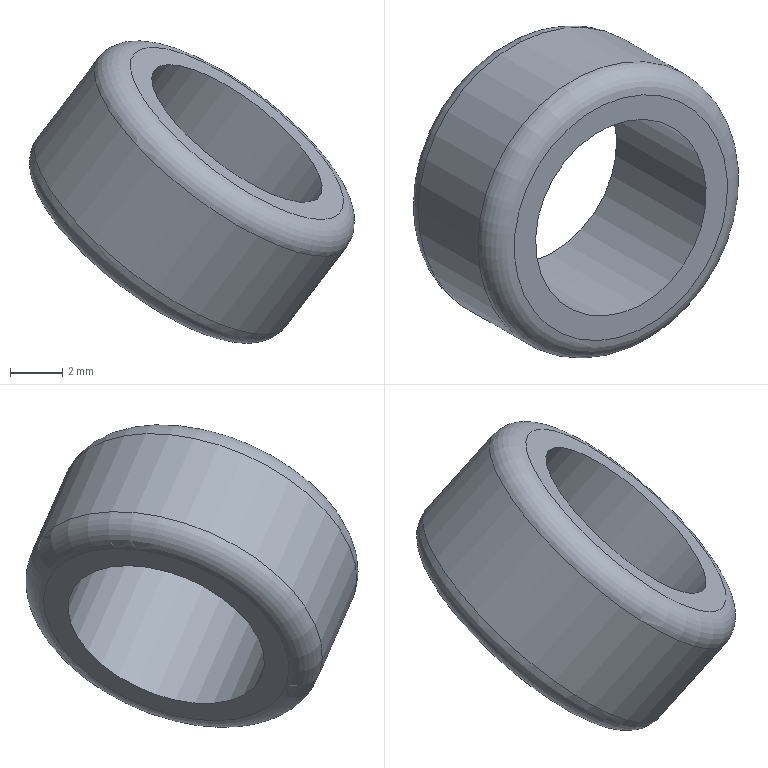Component | NX | YUAN_HUAN_KUAI | 1 solid | 6 faces | volume 361 mm3 | cylinder 2 | plane 2 | torus 2 | commonest cylinder face diameters 12 x1 8 x1
STEP:
#1=CARTESIAN_POINT('',(0.,0.,0.));
#2=DIRECTION('',(0.,0.,1.));
#3=DIRECTION('',(1.,0.,0.));
#4=AXIS2_PLACEMENT_3D('',#1,#2,#3);
#5=CARTESIAN_POINT('',(-203.835,-46.755,66.676));
#6=VERTEX_POINT('',#5);
#7=CARTESIAN_POINT('',(-201.952,-41.152,67.703));
#8=DIRECTION('',(0.5736,-0.3301,0.7497));
#9=DIRECTION('',(-0.3138,-0.9339,-0.1711));
#10=AXIS2_PLACEMENT_3D('',#7,#8,#9);
#11=CIRCLE('',#10,6.);
#12=CARTESIAN_POINT('',(-199.085,-42.802,71.452));
#13=DIRECTION('',(-0.5736,0.3301,-0.7497));
#14=DIRECTION('',(0.3138,0.9339,0.1711));
#15=AXIS2_PLACEMENT_3D('',#12,#13,#14);
#16=CYLINDRICAL_SURFACE('',#15,6.);
#17=CARTESIAN_POINT('',(9.425,5.));
#18=DIRECTION('',(-1.,0.));
#19=VECTOR('',#18,1.);
#20=LINE('',#17,#19);
#21=(GEOMETRIC_REPRESENTATION_CONTEXT(2)PARAMETRIC_REPRESENTATION_CONTEXT()REPRESENTATION_CONTEXT('',''));
#22=DEFINITIONAL_REPRESENTATION('',(#20),#21);
#23=PCURVE('',#16,#22);
#24=CARTESIAN_POINT('',(-201.952,-41.152,67.703));
#25=DIRECTION('',(0.5736,-0.3301,0.7497));
#26=DIRECTION('',(-0.3138,-0.9339,-0.1711));
#27=AXIS2_PLACEMENT_3D('',#24,#25,#26);
#28=TOROIDAL_SURFACE('',#27,5.,1.);
#29=CARTESIAN_POINT('',(0.,6.283));
#30=DIRECTION('',(1.,0.));
#31=VECTOR('',#30,1.);
#32=LINE('',#29,#31);
#33=(GEOMETRIC_REPRESENTATION_CONTEXT(2)PARAMETRIC_REPRESENTATION_CONTEXT()REPRESENTATION_CONTEXT('',''));
#34=DEFINITIONAL_REPRESENTATION('',(#32),#33);
#35=PCURVE('',#28,#34);
#36=SURFACE_CURVE('',#11,(#23,#35),.PCURVE_S1.);
#37=EDGE_CURVE('',#6,#6,#36,.T.);
#38=ORIENTED_EDGE('',*,*,#37,.T.);
#39=CARTESIAN_POINT('',(-201.541,-48.076,69.675));
#40=VERTEX_POINT('',#39);
#41=CARTESIAN_POINT('',(-201.541,-48.076,69.675));
#42=CARTESIAN_POINT('',(-203.835,-46.755,66.676));
#43=B_SPLINE_CURVE_WITH_KNOTS('',1,(#41,#42),.UNSPECIFIED.,.F.,.F.,(2,2),(1.,5.),.PIECEWISE_BEZIER_KNOTS.);
#44=CARTESIAN_POINT('',(3.142,0.));
#45=DIRECTION('',(0.,1.));
#46=VECTOR('',#45,1.);
#47=LINE('',#44,#46);
#48=(GEOMETRIC_REPRESENTATION_CONTEXT(2)PARAMETRIC_REPRESENTATION_CONTEXT()REPRESENTATION_CONTEXT('',''));
#49=DEFINITIONAL_REPRESENTATION('',(#47),#48);
#50=PCURVE('',#16,#49);
#51=CARTESIAN_POINT('',(9.425,0.));
#52=DIRECTION('',(0.,1.));
#53=VECTOR('',#52,1.);
#54=LINE('',#51,#53);
#55=(GEOMETRIC_REPRESENTATION_CONTEXT(2)PARAMETRIC_REPRESENTATION_CONTEXT()REPRESENTATION_CONTEXT('',''));
#56=DEFINITIONAL_REPRESENTATION('',(#54),#55);
#57=PCURVE('',#16,#56);
#58=SEAM_CURVE('',#43,(#50,#57),.PCURVE_S1.);
#59=EDGE_CURVE('',#40,#6,#58,.T.);
#60=ORIENTED_EDGE('',*,*,#59,.F.);
#61=CARTESIAN_POINT('',(-199.658,-42.472,70.702));
#62=DIRECTION('',(-0.5736,0.3301,-0.7497));
#63=DIRECTION('',(-0.3138,-0.9339,-0.1711));
#64=AXIS2_PLACEMENT_3D('',#61,#62,#63);
#65=CIRCLE('',#64,6.);
#66=CARTESIAN_POINT('',(3.142,1.));
#67=DIRECTION('',(1.,0.));
#68=VECTOR('',#67,1.);
#69=LINE('',#66,#68);
#70=(GEOMETRIC_REPRESENTATION_CONTEXT(2)PARAMETRIC_REPRESENTATION_CONTEXT()REPRESENTATION_CONTEXT('',''));
#71=DEFINITIONAL_REPRESENTATION('',(#69),#70);
#72=PCURVE('',#16,#71);
#73=CARTESIAN_POINT('',(-199.658,-42.472,70.702));
#74=DIRECTION('',(0.5736,-0.3301,0.7497));
#75=DIRECTION('',(-0.3138,-0.9339,-0.1711));
#76=AXIS2_PLACEMENT_3D('',#73,#74,#75);
#77=TOROIDAL_SURFACE('',#76,5.,1.);
#78=CARTESIAN_POINT('',(6.283,6.283));
#79=CARTESIAN_POINT('',(6.188,6.283));
#80=CARTESIAN_POINT('',(5.998,6.283));
#81=CARTESIAN_POINT('',(5.712,6.283));
#82=CARTESIAN_POINT('',(5.426,6.283));
#83=CARTESIAN_POINT('',(5.141,6.283));
#84=CARTESIAN_POINT('',(4.855,6.283));
#85=CARTESIAN_POINT('',(4.57,6.283));
#86=CARTESIAN_POINT('',(4.284,6.283));
#87=CARTESIAN_POINT('',(3.998,6.283));
#88=CARTESIAN_POINT('',(3.713,6.283));
#89=CARTESIAN_POINT('',(3.427,6.283));
#90=CARTESIAN_POINT('',(3.142,6.283));
#91=CARTESIAN_POINT('',(2.856,6.283));
#92=CARTESIAN_POINT('',(2.57,6.283));
#93=CARTESIAN_POINT('',(2.285,6.283));
#94=CARTESIAN_POINT('',(1.999,6.283));
#95=CARTESIAN_POINT('',(1.714,6.283));
#96=CARTESIAN_POINT('',(1.428,6.283));
#97=CARTESIAN_POINT('',(1.142,6.283));
#98=CARTESIAN_POINT('',(0.8568,6.283));
#99=CARTESIAN_POINT('',(0.5712,6.283));
#100=CARTESIAN_POINT('',(0.2856,6.283));
#101=CARTESIAN_POINT('',(0.0952,6.283));
#102=CARTESIAN_POINT('',(0.,6.283));
#103=B_SPLINE_CURVE_WITH_KNOTS('',3,(#78,#79,#80,#81,#82,#83,#84,#85,#86,#87,#88,#89,#90,#91,#92,#93,#94,#95,#96,#97,#98,#99,#100,#101,#102),.UNSPECIFIED.,.F.,.F.,(4,1,1,1,1,1,1,1,1,1,1,1,1,1,1,1,1,1,1,1,1,1,4),(0.,0.2856,0.5712,0.8568,1.142,1.428,1.714,1.999,2.285,2.57,2.856,3.142,3.427,3.713,3.998,4.284,4.57,4.855,5.141,5.426,5.712,5.998,6.283),.QUASI_UNIFORM_KNOTS.);
#104=(GEOMETRIC_REPRESENTATION_CONTEXT(2)PARAMETRIC_REPRESENTATION_CONTEXT()REPRESENTATION_CONTEXT('',''));
#105=DEFINITIONAL_REPRESENTATION('',(#103),#104);
#106=PCURVE('',#77,#105);
#107=SURFACE_CURVE('',#65,(#72,#106),.PCURVE_S1.);
#108=EDGE_CURVE('',#40,#40,#107,.T.);
#109=ORIENTED_EDGE('',*,*,#108,.T.);
#110=ORIENTED_EDGE('',*,*,#59,.T.);
#111=EDGE_LOOP('',(#38,#60,#109,#110));
#112=FACE_BOUND('',#111,.T.);
#113=ADVANCED_FACE('',(#112),#16,.T.);
#114=CARTESIAN_POINT('',(-200.34,-46.538,70.767));
#115=VERTEX_POINT('',#114);
#116=CARTESIAN_POINT('',(-199.085,-42.802,71.452));
#117=DIRECTION('',(0.5736,-0.3301,0.7497));
#118=DIRECTION('',(-0.3138,-0.9339,-0.1711));
#119=AXIS2_PLACEMENT_3D('',#116,#117,#118);
#120=CIRCLE('',#119,4.);
#121=CARTESIAN_POINT('',(-199.085,-42.802,71.452));
#122=DIRECTION('',(-0.5736,0.3301,-0.7497));
#123=DIRECTION('',(0.3138,0.9339,0.1711));
#124=AXIS2_PLACEMENT_3D('',#121,#122,#123);
#125=CYLINDRICAL_SURFACE('',#124,4.);
#126=CARTESIAN_POINT('',(9.425,0.));
#127=DIRECTION('',(-1.,0.));
#128=VECTOR('',#127,1.);
#129=LINE('',#126,#128);
#130=(GEOMETRIC_REPRESENTATION_CONTEXT(2)PARAMETRIC_REPRESENTATION_CONTEXT()REPRESENTATION_CONTEXT('',''));
#131=DEFINITIONAL_REPRESENTATION('',(#129),#130);
#132=PCURVE('',#125,#131);
#133=CARTESIAN_POINT('',(-199.085,-42.802,71.452));
#134=DIRECTION('',(0.5736,-0.3301,0.7497));
#135=DIRECTION('',(-0.3138,-0.9339,-0.1711));
#136=AXIS2_PLACEMENT_3D('',#133,#134,#135);
#137=PLANE('',#136);
#138=CARTESIAN_POINT('',(0.,0.));
#139=DIRECTION('',(1.,0.));
#140=AXIS2_PLACEMENT_2D('',#138,#139);
#141=CIRCLE('',#140,4.);
#142=(GEOMETRIC_REPRESENTATION_CONTEXT(2)PARAMETRIC_REPRESENTATION_CONTEXT()REPRESENTATION_CONTEXT('',''));
#143=DEFINITIONAL_REPRESENTATION('',(#141),#142);
#144=PCURVE('',#137,#143);
#145=SURFACE_CURVE('',#120,(#132,#144),.PCURVE_S1.);
#146=EDGE_CURVE('',#115,#115,#145,.T.);
#147=ORIENTED_EDGE('',*,*,#146,.F.);
#148=CARTESIAN_POINT('',(-203.781,-44.557,66.269));
#149=VERTEX_POINT('',#148);
#150=CARTESIAN_POINT('',(-200.34,-46.538,70.767));
#151=CARTESIAN_POINT('',(-203.781,-44.557,66.269));
#152=B_SPLINE_CURVE_WITH_KNOTS('',1,(#150,#151),.UNSPECIFIED.,.F.,.F.,(2,2),(0.,6.),.PIECEWISE_BEZIER_KNOTS.);
#153=CARTESIAN_POINT('',(9.425,0.));
#154=DIRECTION('',(0.,1.));
#155=VECTOR('',#154,1.);
#156=LINE('',#153,#155);
#157=(GEOMETRIC_REPRESENTATION_CONTEXT(2)PARAMETRIC_REPRESENTATION_CONTEXT()REPRESENTATION_CONTEXT('',''));
#158=DEFINITIONAL_REPRESENTATION('',(#156),#157);
#159=PCURVE('',#125,#158);
#160=CARTESIAN_POINT('',(3.142,0.));
#161=DIRECTION('',(0.,1.));
#162=VECTOR('',#161,1.);
#163=LINE('',#160,#162);
#164=(GEOMETRIC_REPRESENTATION_CONTEXT(2)PARAMETRIC_REPRESENTATION_CONTEXT()REPRESENTATION_CONTEXT('',''));
#165=DEFINITIONAL_REPRESENTATION('',(#163),#164);
#166=PCURVE('',#125,#165);
#167=SEAM_CURVE('',#152,(#159,#166),.PCURVE_S1.);
#168=EDGE_CURVE('',#115,#149,#167,.T.);
#169=ORIENTED_EDGE('',*,*,#168,.T.);
#170=CARTESIAN_POINT('',(-202.526,-40.822,66.954));
#171=DIRECTION('',(0.5736,-0.3301,0.7497));
#172=DIRECTION('',(-0.3138,-0.9339,-0.1711));
#173=AXIS2_PLACEMENT_3D('',#170,#171,#172);
#174=CIRCLE('',#173,4.);
#175=CARTESIAN_POINT('',(9.425,6.));
#176=DIRECTION('',(-1.,0.));
#177=VECTOR('',#176,1.);
#178=LINE('',#175,#177);
#179=(GEOMETRIC_REPRESENTATION_CONTEXT(2)PARAMETRIC_REPRESENTATION_CONTEXT()REPRESENTATION_CONTEXT('',''));
#180=DEFINITIONAL_REPRESENTATION('',(#178),#179);
#181=PCURVE('',#125,#180);
#182=CARTESIAN_POINT('',(-202.526,-40.822,66.954));
#183=DIRECTION('',(0.5736,-0.3301,0.7497));
#184=DIRECTION('',(-0.3138,-0.9339,-0.1711));
#185=AXIS2_PLACEMENT_3D('',#182,#183,#184);
#186=PLANE('',#185);
#187=CARTESIAN_POINT('',(0.,0.));
#188=DIRECTION('',(1.,0.));
#189=AXIS2_PLACEMENT_2D('',#187,#188);
#190=CIRCLE('',#189,4.);
#191=(GEOMETRIC_REPRESENTATION_CONTEXT(2)PARAMETRIC_REPRESENTATION_CONTEXT()REPRESENTATION_CONTEXT('',''));
#192=DEFINITIONAL_REPRESENTATION('',(#190),#191);
#193=PCURVE('',#186,#192);
#194=SURFACE_CURVE('',#174,(#181,#193),.PCURVE_S1.);
#195=EDGE_CURVE('',#149,#149,#194,.T.);
#196=ORIENTED_EDGE('',*,*,#195,.T.);
#197=ORIENTED_EDGE('',*,*,#168,.F.);
#198=EDGE_LOOP('',(#147,#169,#196,#197));
#199=FACE_BOUND('',#198,.F.);
#200=ADVANCED_FACE('',(#199),#125,.F.);
#201=CARTESIAN_POINT('',(-200.653,-47.472,70.596));
#202=VERTEX_POINT('',#201);
#203=CARTESIAN_POINT('',(-199.085,-42.802,71.452));
#204=DIRECTION('',(0.5736,-0.3301,0.7497));
#205=DIRECTION('',(-0.3138,-0.9339,-0.1711));
#206=AXIS2_PLACEMENT_3D('',#203,#204,#205);
#207=CIRCLE('',#206,5.);
#208=CARTESIAN_POINT('',(0.,0.));
#209=DIRECTION('',(1.,-0.));
#210=AXIS2_PLACEMENT_2D('',#208,#209);
#211=CIRCLE('',#210,5.);
#212=(GEOMETRIC_REPRESENTATION_CONTEXT(2)PARAMETRIC_REPRESENTATION_CONTEXT()REPRESENTATION_CONTEXT('',''));
#213=DEFINITIONAL_REPRESENTATION('',(#211),#212);
#214=PCURVE('',#137,#213);
#215=CARTESIAN_POINT('',(0.,7.854));
#216=DIRECTION('',(1.,0.));
#217=VECTOR('',#216,1.);
#218=LINE('',#215,#217);
#219=(GEOMETRIC_REPRESENTATION_CONTEXT(2)PARAMETRIC_REPRESENTATION_CONTEXT()REPRESENTATION_CONTEXT('',''));
#220=DEFINITIONAL_REPRESENTATION('',(#218),#219);
#221=PCURVE('',#77,#220);
#222=SURFACE_CURVE('',#207,(#214,#221),.PCURVE_S1.);
#223=EDGE_CURVE('',#202,#202,#222,.T.);
#224=ORIENTED_EDGE('',*,*,#223,.T.);
#225=EDGE_LOOP('',(#224));
#226=FACE_BOUND('',#225,.T.);
#227=ORIENTED_EDGE('',*,*,#146,.F.);
#228=EDGE_LOOP('',(#227));
#229=FACE_BOUND('',#228,.T.);
#230=ADVANCED_FACE('',(#226,#229),#137,.T.);
#231=CARTESIAN_POINT('',(-204.095,-45.491,66.098));
#232=VERTEX_POINT('',#231);
#233=CARTESIAN_POINT('',(-202.526,-40.822,66.954));
#234=DIRECTION('',(-0.5736,0.3301,-0.7497));
#235=DIRECTION('',(-0.3138,-0.9339,-0.1711));
#236=AXIS2_PLACEMENT_3D('',#233,#234,#235);
#237=CIRCLE('',#236,5.);
#238=CARTESIAN_POINT('',(5.,-0.));
#239=CARTESIAN_POINT('',(5.,-8.66));
#240=CARTESIAN_POINT('',(-2.5,-4.33));
#241=CARTESIAN_POINT('',(-10.,0.));
#242=CARTESIAN_POINT('',(-2.5,4.33));
#243=CARTESIAN_POINT('',(5.,8.66));
#244=CARTESIAN_POINT('',(5.,-0.));
#245=(BOUNDED_CURVE()B_SPLINE_CURVE(2,(#238,#239,#240,#241,#242,#243,#244),.UNSPECIFIED.,.T.,.F.)B_SPLINE_CURVE_WITH_KNOTS((1,2,2,2,2,1),(-2.094,0.,2.094,4.189,6.283,8.378),.UNSPECIFIED.)CURVE()GEOMETRIC_REPRESENTATION_ITEM()RATIONAL_B_SPLINE_CURVE((1.,0.5,1.,0.5,1.,0.5,1.))REPRESENTATION_ITEM(''));
#246=(GEOMETRIC_REPRESENTATION_CONTEXT(2)PARAMETRIC_REPRESENTATION_CONTEXT()REPRESENTATION_CONTEXT('',''));
#247=DEFINITIONAL_REPRESENTATION('',(#245),#246);
#248=PCURVE('',#186,#247);
#249=CARTESIAN_POINT('',(6.283,4.712));
#250=DIRECTION('',(-1.,0.));
#251=VECTOR('',#250,1.);
#252=LINE('',#249,#251);
#253=(GEOMETRIC_REPRESENTATION_CONTEXT(2)PARAMETRIC_REPRESENTATION_CONTEXT()REPRESENTATION_CONTEXT('',''));
#254=DEFINITIONAL_REPRESENTATION('',(#252),#253);
#255=PCURVE('',#28,#254);
#256=SURFACE_CURVE('',#237,(#248,#255),.PCURVE_S1.);
#257=EDGE_CURVE('',#232,#232,#256,.T.);
#258=ORIENTED_EDGE('',*,*,#257,.T.);
#259=EDGE_LOOP('',(#258));
#260=FACE_BOUND('',#259,.T.);
#261=ORIENTED_EDGE('',*,*,#195,.T.);
#262=EDGE_LOOP('',(#261));
#263=FACE_BOUND('',#262,.T.);
#264=ADVANCED_FACE('',(#260,#263),#186,.F.);
#265=ORIENTED_EDGE('',*,*,#257,.F.);
#266=CARTESIAN_POINT('',(-204.095,-45.491,66.098));
#267=CARTESIAN_POINT('',(-204.179,-45.741,66.052));
#268=CARTESIAN_POINT('',(-204.212,-46.012,66.071));
#269=CARTESIAN_POINT('',(-204.189,-46.276,66.155));
#270=CARTESIAN_POINT('',(-204.111,-46.502,66.295));
#271=CARTESIAN_POINT('',(-203.988,-46.667,66.476));
#272=CARTESIAN_POINT('',(-203.835,-46.755,66.676));
#273=(BOUNDED_CURVE()B_SPLINE_CURVE(6,(#266,#267,#268,#269,#270,#271,#272),.UNSPECIFIED.,.F.,.F.)B_SPLINE_CURVE_WITH_KNOTS((7,7),(4.712,6.283),.PIECEWISE_BEZIER_KNOTS.)CURVE()GEOMETRIC_REPRESENTATION_ITEM()RATIONAL_B_SPLINE_CURVE((1.031,1.01,0.9979,0.994,0.9979,1.01,1.031))REPRESENTATION_ITEM(''));
#274=CARTESIAN_POINT('',(6.283,0.));
#275=DIRECTION('',(0.,1.));
#276=VECTOR('',#275,1.);
#277=LINE('',#274,#276);
#278=(GEOMETRIC_REPRESENTATION_CONTEXT(2)PARAMETRIC_REPRESENTATION_CONTEXT()REPRESENTATION_CONTEXT('',''));
#279=DEFINITIONAL_REPRESENTATION('',(#277),#278);
#280=PCURVE('',#28,#279);
#281=CARTESIAN_POINT('',(0.,0.));
#282=DIRECTION('',(0.,1.));
#283=VECTOR('',#282,1.);
#284=LINE('',#281,#283);
#285=(GEOMETRIC_REPRESENTATION_CONTEXT(2)PARAMETRIC_REPRESENTATION_CONTEXT()REPRESENTATION_CONTEXT('',''));
#286=DEFINITIONAL_REPRESENTATION('',(#284),#285);
#287=PCURVE('',#28,#286);
#288=SEAM_CURVE('',#273,(#280,#287),.PCURVE_S1.);
#289=EDGE_CURVE('',#232,#6,#288,.T.);
#290=ORIENTED_EDGE('',*,*,#289,.T.);
#291=ORIENTED_EDGE('',*,*,#37,.F.);
#292=ORIENTED_EDGE('',*,*,#289,.F.);
#293=EDGE_LOOP('',(#265,#290,#291,#292));
#294=FACE_BOUND('',#293,.T.);
#295=ADVANCED_FACE('',(#294),#28,.T.);
#296=ORIENTED_EDGE('',*,*,#108,.F.);
#297=CARTESIAN_POINT('',(-201.541,-48.076,69.675));
#298=CARTESIAN_POINT('',(-201.387,-48.164,69.876));
#299=CARTESIAN_POINT('',(-201.211,-48.171,70.085));
#300=CARTESIAN_POINT('',(-201.032,-48.092,70.281));
#301=CARTESIAN_POINT('',(-200.868,-47.937,70.442));
#302=CARTESIAN_POINT('',(-200.737,-47.722,70.55));
#303=CARTESIAN_POINT('',(-200.653,-47.472,70.596));
#304=(BOUNDED_CURVE()B_SPLINE_CURVE(6,(#297,#298,#299,#300,#301,#302,#303),.UNSPECIFIED.,.F.,.F.)B_SPLINE_CURVE_WITH_KNOTS((7,7),(0.,1.571),.PIECEWISE_BEZIER_KNOTS.)CURVE()GEOMETRIC_REPRESENTATION_ITEM()RATIONAL_B_SPLINE_CURVE((1.031,1.01,0.9979,0.994,0.9979,1.01,1.031))REPRESENTATION_ITEM(''));
#305=CARTESIAN_POINT('',(6.283,6.283));
#306=DIRECTION('',(0.,1.));
#307=VECTOR('',#306,1.);
#308=LINE('',#305,#307);
#309=(GEOMETRIC_REPRESENTATION_CONTEXT(2)PARAMETRIC_REPRESENTATION_CONTEXT()REPRESENTATION_CONTEXT('',''));
#310=DEFINITIONAL_REPRESENTATION('',(#308),#309);
#311=PCURVE('',#77,#310);
#312=CARTESIAN_POINT('',(0.,6.283));
#313=DIRECTION('',(0.,1.));
#314=VECTOR('',#313,1.);
#315=LINE('',#312,#314);
#316=(GEOMETRIC_REPRESENTATION_CONTEXT(2)PARAMETRIC_REPRESENTATION_CONTEXT()REPRESENTATION_CONTEXT('',''));
#317=DEFINITIONAL_REPRESENTATION('',(#315),#316);
#318=PCURVE('',#77,#317);
#319=SEAM_CURVE('',#304,(#311,#318),.PCURVE_S1.);
#320=EDGE_CURVE('',#40,#202,#319,.T.);
#321=ORIENTED_EDGE('',*,*,#320,.T.);
#322=ORIENTED_EDGE('',*,*,#223,.F.);
#323=ORIENTED_EDGE('',*,*,#320,.F.);
#324=EDGE_LOOP('',(#296,#321,#322,#323));
#325=FACE_BOUND('',#324,.T.);
#326=ADVANCED_FACE('',(#325),#77,.T.);
#327=CLOSED_SHELL('',(#113,#200,#230,#264,#295,#326));
#328=MANIFOLD_SOLID_BREP('',#327);
#329=(LENGTH_UNIT()NAMED_UNIT(*)SI_UNIT(.MILLI.,.METRE.));
#330=UNCERTAINTY_MEASURE_WITH_UNIT(LENGTH_MEASURE(0.00001),#329,'','');
#331=(NAMED_UNIT(*)PLANE_ANGLE_UNIT()SI_UNIT($,.RADIAN.));
#332=(NAMED_UNIT(*)SI_UNIT($,.STERADIAN.)SOLID_ANGLE_UNIT());
#333=(GEOMETRIC_REPRESENTATION_CONTEXT(3)GLOBAL_UNCERTAINTY_ASSIGNED_CONTEXT((#330))GLOBAL_UNIT_ASSIGNED_CONTEXT((#329,#331,#332))REPRESENTATION_CONTEXT('',''));
#334=ADVANCED_BREP_SHAPE_REPRESENTATION('',(#4,#328),#333);